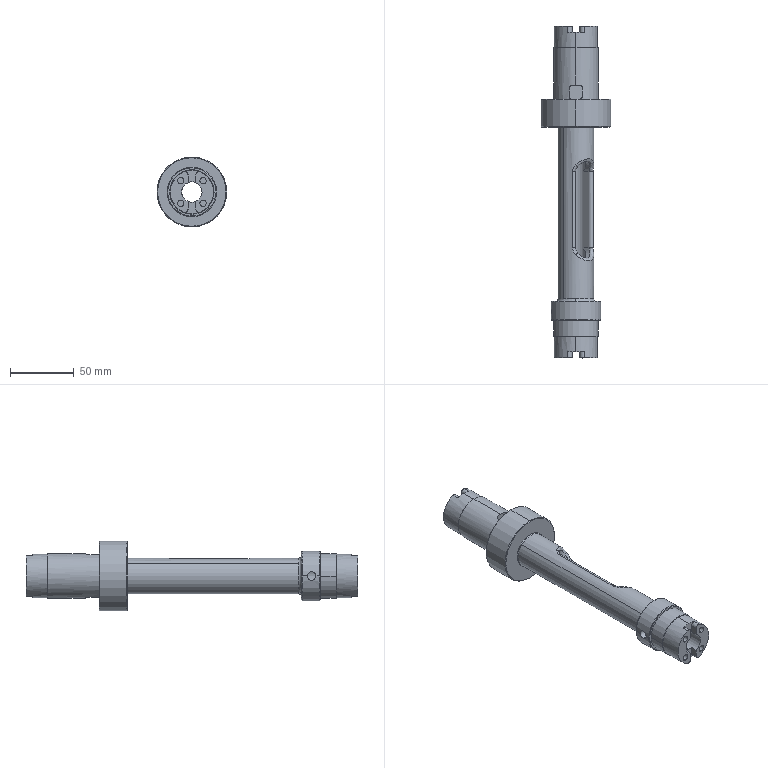CAM job | Mastercam | mm | 6 operations | part box 55 x 261 x 55
1. Drill/Counterbore | 7 - 4 倒角刀
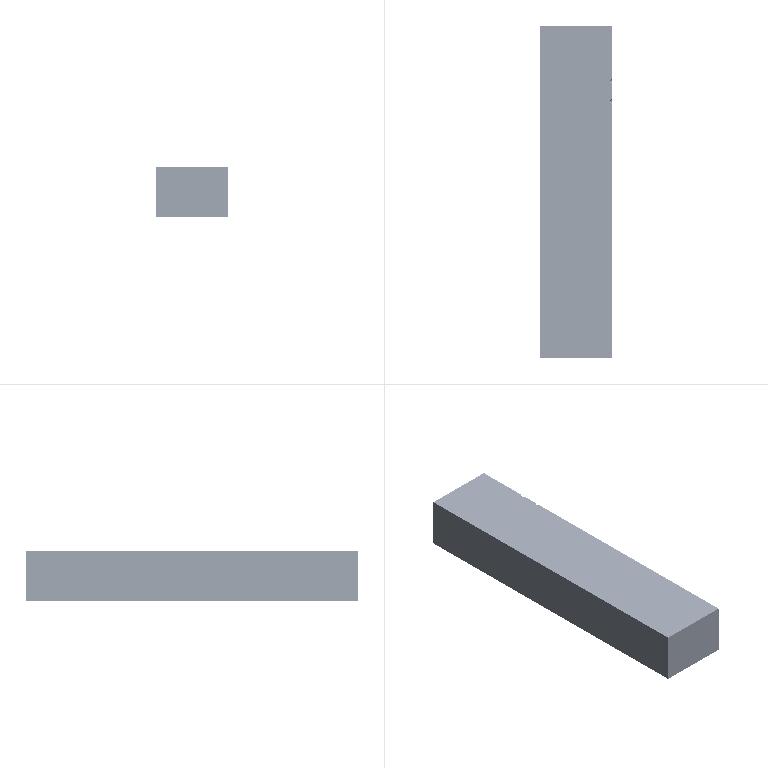2. Peck Drill | 1 - 2.5 钻头
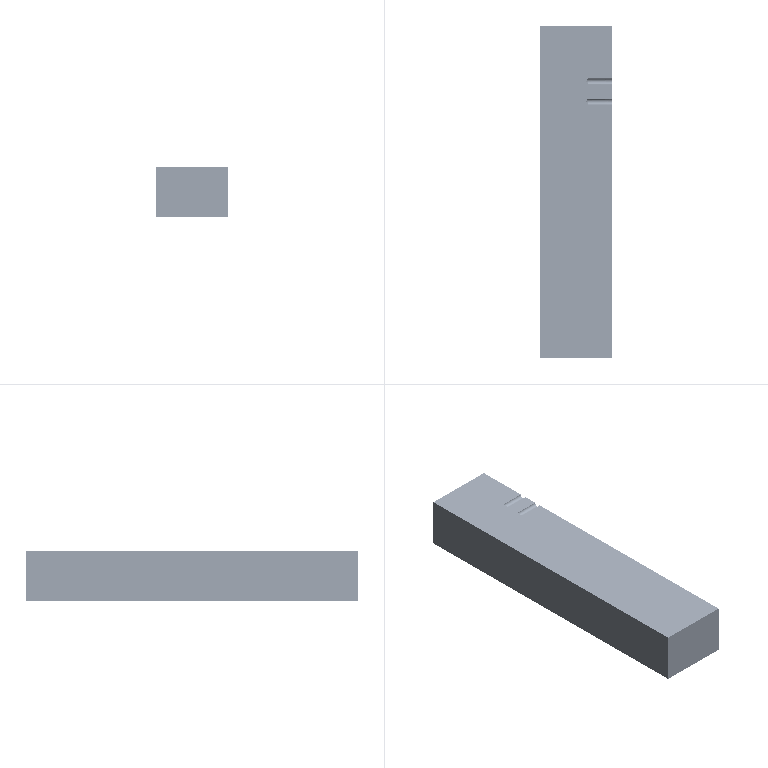3. Drill/Counterbore | 7 - 4 倒角刀
4. Peck Drill | 1 - 6.9 钻头
5. 3D High Speed (Area roughing) | 10 - 10 平铣刀
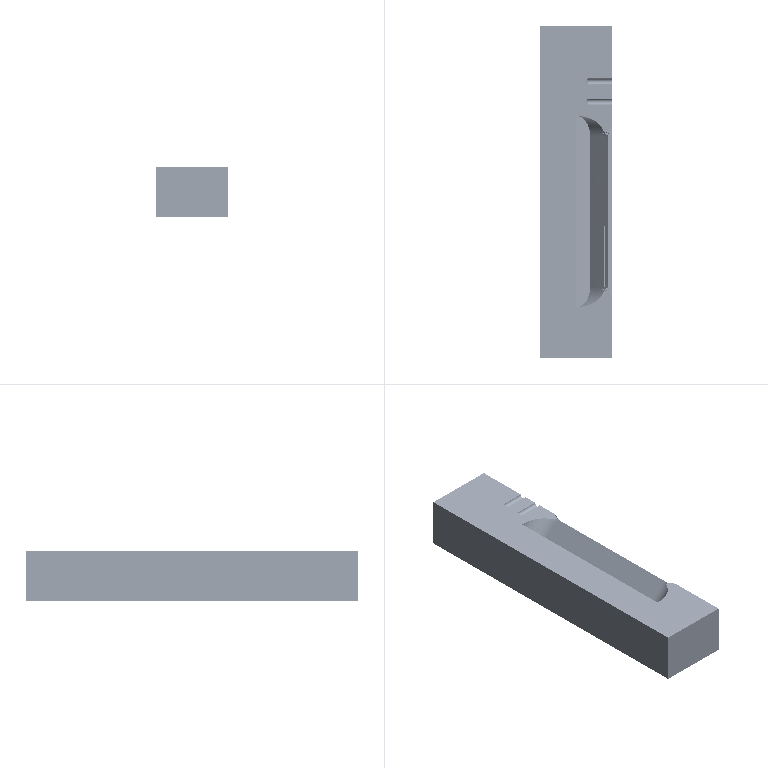6. Unified Morph | 5 - 6 球刀/圆鼻铣刀